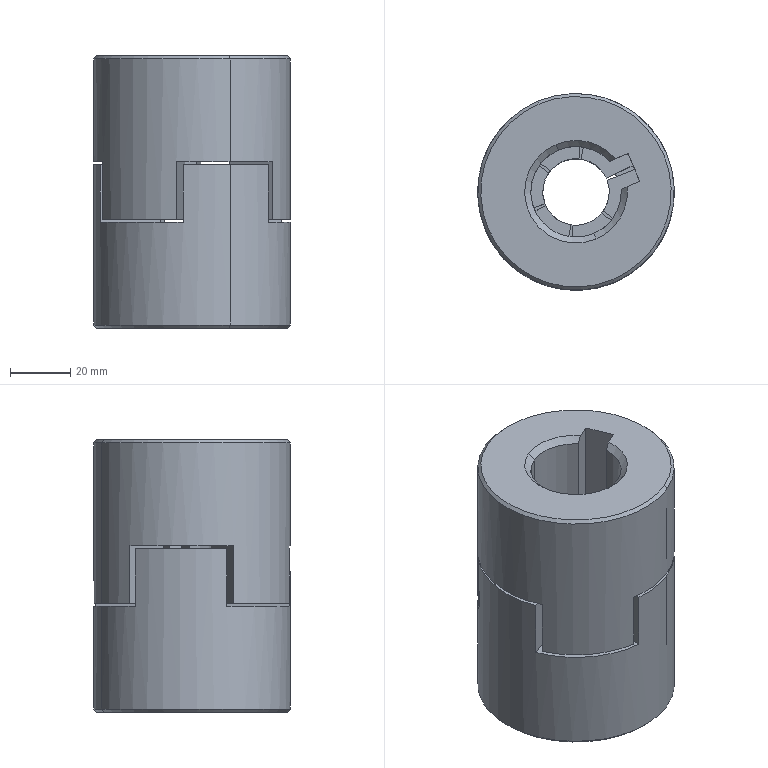Component | SolidWorks | XLJ2-22-22-1 | 2 solids | 72 faces | volume 241080 mm3 | plane 44 | cylinder 18 | cone 10 | commonest cylinder face diameters 30 x7 22 x7 65 x4 | material Plain Carbon Steel